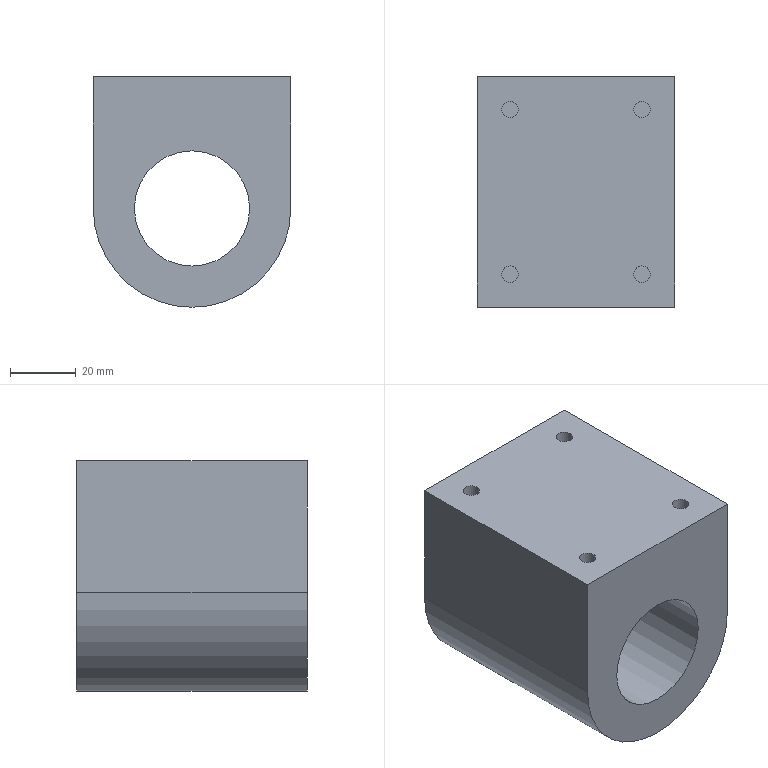Component | NX | SLEEVE_2 | 1 solid | 23 faces | volume 194986 mm3 | cylinder 10 | plane 9 | cone 4 | commonest cylinder face diameters 5 x4 6.8 x4 60 x1 35 x1